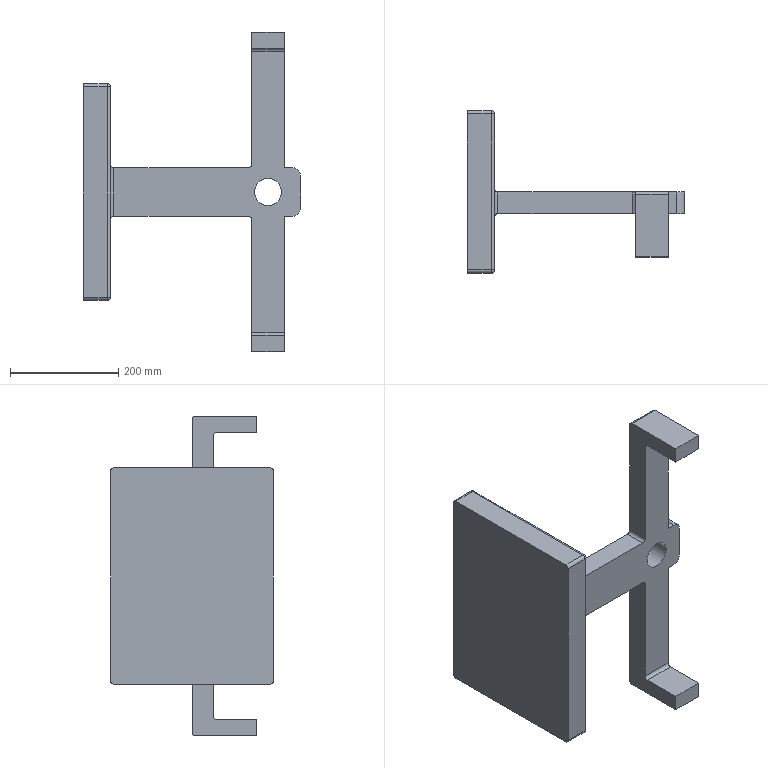Component | NX | SIRT | 1 solid | 48 faces | volume 8658610 mm3 | plane 23 | cylinder 21 | sphere 4 | commonest cylinder face diameters 12 x18 30 x1 30.273 x1 50 x1